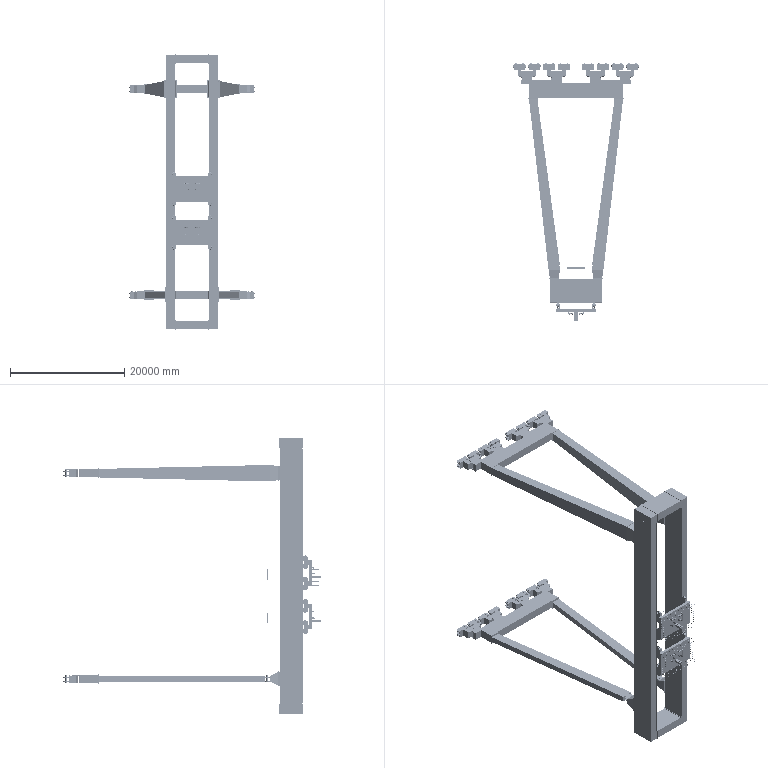Assembly | SolidWorks | mm | 212 component files | 216 solids | 10442 faces | box 22000.01 x 45009.52 x 48200 mm | volume 247326678833 mm3 | plane 6096 | cylinder 3432 | torus 512 | spline 402 | commonest cylinder face diameters 40 x1936 300 x592 200 x396 1000 x192 160 x88 80 x48 10 x32 700 x32
Bill of materials:
EndBeam | 2 |  | Rectangular box-shaped enclosure with a solid top and sides, and a thin plate at each end that sticks out a little past the body outline. One end plate has a row of small holes around its edge and a rounded-rectangle cutout in the middle.
FlexibleLegGenuine | 2 |  | Long, straight beam with a rectangular cross-section. One end has a wider rectangular plate with holes around its edge. The other end has two parallel flat tabs with rounded ends and a hole in each, like a clevis.
FlexibleLegPinAxis | 2 |  | Plain solid cylinder with flat ends.
FlexibleLegSaddleBody | 2 |  | Tapered transition body. The large end is a flat rectangular flange with holes around its edge and a rounded-rectangle opening. The body narrows to the other end, which carries three parallel lug plates with rounded tops and a through hole, like a multi-tab clevis.
16 | 2 |  | Thin, flat rectangular plate or panel with a few small slots and tabs near its centre. A wireframe-only rectangular box with evenly spaced cross lines sits on one side of it.
18 | 4 |  | Solid rectangular bar with a slightly larger, thin rectangular plate at one end.
20 | 8 |  | Clevis- or fork-shaped part: two parallel flat side plates with rounded ends, joined by a cross pin near the rounded end. The other end of the plates attaches to a flat rectangular base plate.
21 | 2 |  | Flat rectangular panel with narrow upright end strips. The strips run the full height and stick out past the panel on one face and at the top and bottom.
22 | 4 |  | Cylindrical roller or tube with a flanged collar near each end. An arm on each end runs out sideways and ends in a small rectangular block. From the end, one side is round and the other is a straight arm with a widened tip, like a keyhole.
27 | 2 |  | Wire form with two side-by-side helical coil sections joined by a U-shaped loop. A long straight leg runs from each coil and ends in a small coiled end, like a double torsion spring.
28 | 2 |  | Wire form with two side-by-side helical coil sections joined by a U-shaped loop. A long straight leg runs from each coil and ends in a small coiled end, like a double torsion spring.
Part15 | 16 |  | Grooved disc, like a pulley or spool: a short cylinder with a centre bore and a deep groove around its outside between two equal side flanges.
Part16 | 8 |  | Thin-walled U-channel bracket with two parallel side walls joined by a base web; one wall carries two round through-holes and a raised rectangular block or step on the outer face of the web.
Part17 | 16 |  | Plain solid cylinder (round rod segment) with flat ends.
LowerCrossbeam | 2 |  | Long straight rectangular box-section body with a thin flange plate at each end; each flange has a row of small holes around its edge and a U-shaped raised or recessed feature on its face.
MainBeam | 2 |  | Tall, slender rectangular bar or plate with small steps, tabs or notches along its long edges and near its ends.
RigidLeg | 2 |  | Long hollow rectangular duct section that tapers along its length, with a flat flange at each end; the flanges have perimeter holes and the larger end shows nested internal walls or vanes.
RigidLegSaddleBody | 2 |  | Short, flanged, hollow rectangular transition piece with tapered sides and bolt-hole flanges at both ends; looking through it shows a rounded-rectangle opening crossed by horizontal bars.
10 | 8 |  | Headed cylindrical pin: a plain round shank with a larger, thin, flat circular head at one end.
7 | 8 |  | Solid block with a flat top, vertical sides and a faceted underside (flat bottom with angled faces at each end), with slightly rounded edges and a single vertical round hole at the centre.
9 | 64 |  | Flat annular washer-like ring with a central round hole and rounded outer and inner edges.
Part12 | 16 |  | C-shaped bracket with two parallel flanges extending from a back body: the top flange has two round holes and the lower flange has a visible hole. A rectangular rib on the back body and a short cylindrical boss or pin sticking out at its top and bottom.
Part13 | 4 |  | Elongated thin-walled C-channel bracket with angled, tapered mounting tabs at each end, each tab with one small round hole; the channel has a small step on its underside.
Part14 | 32 |  | Plain solid cylinder (rod or pin) with flat ends, longer than its diameter.
Mates:
1. coincident | MainBeam-1 face at (3551.042, 16068.918, 30073.003) dir (0.0000002, 0, 1) | MainBeam-2 face at (-4068.958, 16068.918, 30073.004) dir (0.0000002, 0, 1)
2. distance | MainBeam-1 face at (2801.042, 18068.918, 30073.003) dir (-1, 0, 0.0000002) | MainBeam-2 face at (-3318.968, 18068.918, -17926.996) dir (1, 0, -0.0000002)
3. coincident | MainBeam-1 face at (4301.042, 18068.918, 30073.003) dir (0, 1, 0) | MainBeam-2 face at (-4818.968, 18068.918, -17926.995) dir (0, 1, 0)
4. width | EndBeam-1 face at (-3158.958, 16068.918, 29323.004) dir (-1, 0, 0.0000002) | EndBeam-1 face at (2641.042, 16068.918, 29323.003) dir (1, 0, -0.0000002) | MainBeam-2 face at (-3318.968, 18068.918, -17926.996) dir (1, 0, -0.0000002) | MainBeam-1 face at (2801.042, 18068.918, 30073.003) dir (-1, 0, 0.0000002)
5. coincident | EndBeam-1 face at (-3143.958, 18068.918, 30073.004) dir (0.0000002, 0, 1) | MainBeam-1 face at (3551.042, 16068.918, 30073.003) dir (0.0000002, 0, 1)
6. coincident | EndBeam-1 face at (-3143.958, 18068.918, 30073.004) dir (0, 1, 0) | MainBeam-1 face at (4301.042, 18068.918, 30073.003) dir (0, 1, 0)
7. coincident | RigidLegSaddleBody-1 face at (-4068.959, 18218.918, 24073.004) dir (0, -1, 0) | MainBeam-2 face at (-4068.963, 18218.918, 6073.004) dir (0, 1, 0)
8. width | RigidLegSaddleBody-1 face at (-3218.96, 18278.918, 22773.004) dir (1, 0, -0.0000002) | RigidLegSaddleBody-1 face at (-4918.959, 18278.918, 25373.005) dir (-1, 0, 0.0000002) | MainBeam-2 face at (-4918.96, 18218.918, 22758.005) dir (-1, 0, 0.0000002) | MainBeam-2 face at (-3218.959, 18218.918, 25388.004) dir (1, 0, -0.0000002)
9. width | RigidLegSaddleBody-1 face at (-3218.959, 18278.918, 25388.004) dir (0.0000002, 0, 1) | RigidLegSaddleBody-1 face at (-4918.96, 18278.918, 22758.005) dir (-0.0000002, 0, -1) | MainBeam-2 face at (-3218.96, 18218.918, 22758.004) dir (-0.0000002, 0, -1) | MainBeam-2 face at (-4918.959, 18218.918, 25388.005) dir (0.0000002, 0, 1)
10. width | RigidLeg-1 face at (-2968.959, 19718.918, 25623.004) dir (0.0000002, 0, 1) | RigidLeg-1 face at (-5168.96, 19718.918, 22523.005) dir (-0.0000002, 0, -1) | RigidLegSaddleBody-1 face at (-2968.96, 19658.918, 22523.004) dir (-0.0000002, 0, -1) | RigidLegSaddleBody-1 face at (-5168.959, 19658.918, 25623.005) dir (0.0000002, 0, 1)
11. width | RigidLeg-1 face at (-5168.959, 19718.918, 25623.005) dir (-1, 0, 0.0000002) | RigidLeg-1 face at (-2968.96, 19718.918, 22523.004) dir (1, 0, -0.0000002) | RigidLegSaddleBody-1 face at (-5168.96, 19658.918, 22523.005) dir (-1, 0, 0.0000002) | RigidLegSaddleBody-1 face at (-2968.959, 19658.918, 25623.004) dir (1, 0, -0.0000002)
12. coincident | RigidLeg-1 face at (-7752.496, 19718.918, 24073.005) dir (0, -1, 0) | RigidLegSaddleBody-1 face at (-4068.959, 19718.918, 24073.004) dir (0, 1, 0)
13. width | FlexibleLegGenuine-2 face at (-7752.504, 49658.918, -12426.995) dir (-0.0000002, 0, -1) | FlexibleLegGenuine-2 face at (-7752.503, 49658.918, -11426.995) dir (0.0000002, 0, 1) | FlexibleLegSaddleBody-1 face at (-4068.967, 18762.883, -12901.694) dir (-0.00000018, 0.4447, -0.8957) | FlexibleLegSaddleBody-1 face at (-4068.966, 18762.883, -10952.297) dir (0.00000018, 0.4447, 0.8957)
14. tangent | FlexibleLegSaddleBody-1 face at (-4068.967, 20018.918, -11506.996) dir (0.0000002, 0, 1) r 600 | FlexibleLegGenuine-2 face at (-7752.503, 20618.918, -11926.995) dir (0, -1, 0)
15. concentric | FlexibleLegSaddleBody-1 edge at (-4068.967, 20198.918, -11966.996) dir (0.0000002, 0, 1) r 200 | FlexibleLegGenuine-2 edge at (-4068.967, 20198.918, -11736.996) dir (-0.0000002, 0, -1) r 200
16. parallel | MainBeam-2 face at (-4068.968, 16068.918, -17926.996) dir (-0.0000002, 0, -1) | FlexibleLegGenuine-2 face at (-7752.504, 49658.918, -12426.995) dir (-0.0000002, 0, -1)
17. parallel | RigidLeg-1 face at (-7752.496, 49718.918, 24073.005) dir (0, 1, 0) | assembly plane at (0, 0, 0) dir (0, 1, 0)
18. coincident | FlexibleLegSaddleBody-1 face at (-4068.967, 18218.918, -11926.996) dir (0, -1, 0) | MainBeam-2 face at (-4068.963, 18218.918, 6073.004) dir (0, 1, 0)
19. width | FlexibleLegSaddleBody-1 face at (-4918.966, 18218.918, -10611.995) dir (-1, 0, 0.0000002) | FlexibleLegSaddleBody-1 face at (-3218.967, 18218.918, -13241.996) dir (1, 0, -0.0000002) | MainBeam-2 face at (-3218.967, 18218.918, -13241.996) dir (1, 0, -0.0000002) | MainBeam-2 face at (-4918.966, 18218.918, -10611.995) dir (-1, 0, 0.0000002)
20. width | FlexibleLegSaddleBody-1 face at (-4918.967, 18218.918, -13241.995) dir (-0.0000002, 0, -1) | FlexibleLegSaddleBody-1 face at (-3218.966, 18218.918, -10611.996) dir (0.0000002, 0, 1) | MainBeam-2 face at (-4918.967, 18218.918, -13241.995) dir (-0.0000002, 0, -1) | MainBeam-2 face at (-3218.966, 18218.918, -10611.996) dir (0.0000002, 0, 1)
21. coincident | FlexibleLegSaddleBody-1 edge at (-4068.967, 20198.918, -12426.996) dir (-0.0000002, 0, -1) r 200 | FlexibleLegPinAxis-1 face at (-4068.967, 20198.918, -12526.996) dir (0.0000002, 0, 1) r 200
22. width | FlexibleLegPinAxis-1 face at (-4068.967, 20198.918, -12526.996) dir (-0.0000002, 0, -1) | FlexibleLegPinAxis-1 face at (-4068.967, 20198.918, -11326.996) dir (0.0000002, 0, 1) | FlexibleLegSaddleBody-1 face at (-5068.967, 19778.918, -11426.995) dir (0.0000002, 0, 1) | FlexibleLegSaddleBody-1 face at (-3068.967, 19778.918, -12426.996) dir (-0.0000002, 0, -1)
23. coincident | RigidLeg-1 face at (-7752.496, 49718.918, 24073.005) dir (0, 1, 0) | LowerCrossbeam-2 face at (-258.959, 49718.918, 24073.004) dir (0, -1, 0)
24. coincident | LowerCrossbeam-2 face at (-8502.494, 52378.918, 24823.005) dir (0, 1, 0) | assembly face at (8891.426, 52779.524, 24005.005) dir (0, -1, 0)
25. width | RunningMechanism-1/7-1 face at (8341.041, 54548.441, 24723.002) dir (0.0000002, 0, 1) | RunningMechanism-1/7-1 face at (8341.04, 54548.441, 23423.002) dir (-0.0000002, 0, -1) | LowerCrossbeam-2 face at (-258.96, 51128.918, 23323.004) dir (-0.0000002, 0, -1) | LowerCrossbeam-2 face at (-258.959, 51128.918, 24823.004) dir (0.0000002, 0, 1)
26. coincident | LowerCrossbeam-2 face at (-8502.494, 52378.918, 24823.005) dir (0, 1, 0) | RunningMechanism-1/Part13-1 face at (5741.04, 52378.918, 23373.003) dir (0, -1, 0)
27. distance | assembly plane at (-258.964, 0, 0.000051) dir (1, 0, -0.0000002) | RunningMechanism-1/Part13-1 face at (4741.04, 52428.918, 23373.003) dir (-1, 0, 0.0000002)
28. tangent | MainBeam-1 face at (2801.042, 13918.918, 30073.003) dir (0, -1, 0) | LiftingAndOperatingMechanism-1/Part15-1 face at (2726.037, 13568.918, 4082.152) dir (-1, 0, 0.0000002) r 350
29. width | LiftingAndOperatingMechanism-1/Part16-1 face at (3126.037, 13443.918, 4782.152) dir (1, 0, -0.0000002) | LiftingAndOperatingMechanism-1/Part16-1 face at (2626.037, 13443.918, 4782.152) dir (-1, 0, 0.0000002) | MainBeam-1 face at (2801.042, 18068.918, 30073.003) dir (-1, 0, 0.0000002) | MainBeam-1 face at (2951.042, 14068.918, 30073.003) dir (1, 0, -0.0000002)
30. parallel | MainBeam-1 face at (4301.042, 14068.918, 30073.003) dir (0, -1, 0) | LiftingAndOperatingMechanism-1/16-1 face at (-258.963, 12918.918, 6632.153) dir (0, 1, 0)
31. width | LiftingAndOperatingMechanism-2/Part16-1 face at (3126.035, 13443.918, -2871.046) dir (1, 0, -0.0000002) | LiftingAndOperatingMechanism-2/Part16-1 face at (2626.035, 13443.918, -2871.046) dir (-1, 0, 0.0000002) | MainBeam-1 face at (2801.042, 18068.918, 30073.003) dir (-1, 0, 0.0000002) | MainBeam-1 face at (2951.042, 14068.918, 30073.003) dir (1, 0, -0.0000002)
32. tangent | MainBeam-2 face at (-3318.968, 13918.918, -17926.996) dir (0, -1, 0) | LiftingAndOperatingMechanism-2/Part15-4 face at (-3243.965, 13568.918, -3571.045) dir (1, 0, -0.0000002) r 350
33. coincident | FlexibleLegGenuine-2 face at (-6902.504, 49718.918, -12776.995) dir (-0.0000002, 0, -1) | LowerCrossbeam-3 face at (-8602.502, 49718.918, -12776.995) dir (-0.0000002, 0, -1)
34. coincident | 16-1 edge at (1000, 480, -300) dir (-1, 0, 0) | 18-2 edge at (1000, 480, -300) dir (-1, 0, 0)
35. coincident | 16-1 edge at (600, 480, -300) dir (0, 0, 1) | 18-2 edge at (600, 480, -300) dir (0, 0, 1)
36. coincident | 16-1 edge at (0, 480, 670) dir (1, 0, 0) | 20-2 edge at (0, 480, 670) dir (1, 0, 0)
37. coincident | 16-1 edge at (200, 480, 670) dir (0, 0, -1) | 20-2 edge at (200, 480, 670) dir (0, 0, -1)
38. coincident | 16-1 edge at (-1000, 480, 1340) dir (1, 0, 0) | 22-1 edge at (-1000, 480, 1340) dir (1, 0, 0)
39. coincident | 16-1 edge at (-1000, 480, 1260) dir (0, 0, 1) | 22-1 edge at (-1000, 480, 1260) dir (0, 0, 1)
40. coincident | 16-1 edge at (430, 480, 1280) dir (1, 0, 0) | 20-1 edge at (280, 480, 1280) dir (1, 0, 0)
41. coincident | 16-1 edge at (480, 480, 1280) dir (0, 0, -1) | 20-1 edge at (480, 480, 1280) dir (0, 0, -1)
42. concentric | 22-1 face at (-900, 820, 520) dir (0, 0, 1) r 130 | 27-1 sketch segment at (-900, 820, 525) dir (0, 0, 1) r 135
43. concentric | 20-1 face at (380, 910, 1255) dir (0, 0, -1) r 40 | 27-1 sketch segment at (380, 910, 525) dir (0, 0, 1) r 45
44. tangent | 22-1 face at (-900, 820, 520) dir (0, 0, 1) | 27-1 face at (-900, 955, 525) dir (1, 0, 0) r 5
45. concentric | 22-2 face at (-900, 820, -1280) dir (0, 0, 1) r 130 | 28-1 sketch segment at (-900, 820, -1225) dir (0, 0, 1) r 135
46. concentric | 20-4 face at (380, 910, -1105) dir (0, 0, -1) r 40 | 28-1 sketch segment at (380, 910, -1225) dir (0, 0, 1) r 45
47. tangent | 22-2 face at (-900, 820, -520) dir (0, 0, -1) | 28-1 face at (-900, 955, -525) dir (1, 0, 0) r 5
48. concentric | 21-1 sketch segment at (144.999, -7090.265, 603.75) dir (0, 1, 0) r 5 | LiftingAndOperatingMechanism sketch segment at (144.999, -7090.265, 603.75) dir (0, -1, 0) r 5
49. concentric | 21-1 sketch segment at (425, -7090.265, 1146.25) dir (0, 1, 0) r 5 | LiftingAndOperatingMechanism sketch segment at (425, -7090.265, 1146.25) dir (0, -1, 0) r 5
50. coincident | 21-1 face at (524.311, -7090.265, -0.000113) dir (0, 1, 0) | LiftingAndOperatingMechanism sketch segment at (425, -7090.265, 1146.25) dir (0, -1, 0) r 5
51. coincident | 16-1 face at (0, 0, 0) dir (0, -1, 0) | Part16-1 face at (1450, 0, -2885) dir (0, 1, 0)
52. coincident | 16-1 face at (2250, 500, -3585) dir (1, 0, 0) | Part16-1 face at (2250, -100, -2885) dir (1, 0, 0)
53. width | Part15-1 face at (2550, -150, -2985) dir (0, 0, 1) | Part15-1 face at (2550, -650, -3285) dir (0, 0, -1) | Part16-1 face at (1850, -525, -3385) dir (0, 0, -1) | Part16-1 face at (1850, -525, -2885) dir (0, 0, 1)
54. concentric | Part15-1 face at (2550, -650, -2985) dir (0, 0, 1) r 500 | Part16-1 face at (2550, -650, -3385) dir (0, 0, 1) r 150
55. distance | Part16-1 face at (1850, -525, -3385) dir (0, 0, -1) | 16-1 face at (-2250, 500, -3585) dir (0, 0, -1)
56. concentric | Part16-1 face at (1150, -650, -3385) dir (0, 0, 1) r 153.74 | Part15-3 face at (1150, -650, -3285) dir (0, 0, -1) r 500
57. width | Part15-3 face at (1150, -1150, -3285) dir (0, 0, -1) | Part15-3 face at (1150, -650, -2985) dir (0, 0, 1) | Part16-1 face at (1850, -525, -2885) dir (0, 0, 1) | Part16-1 face at (1850, -525, -3385) dir (0, 0, -1)
58. concentric | Part16-1 face at (2550, -650, -3385) dir (0, 0, 1) r 150 | Part17-1 face at (2550, -650, -2835) dir (0, 0, -1) r 150
59. width | Part17-1 face at (2550, -650, -2835) dir (0, 0, 1) | Part17-1 face at (2550, -650, -3435) dir (0, 0, -1) | Part16-1 face at (1850, -525, -3385) dir (0, 0, -1) | Part16-1 face at (1850, -525, -2885) dir (0, 0, 1)
60. concentric | Part16-1 face at (1150, -650, -3385) dir (0, 0, 1) r 153.74 | Part17-2 face at (1150, -650, -2835) dir (0, 0, -1) r 150
61. width | Part17-2 face at (1150, -650, -3435) dir (0, 0, -1) | Part17-2 face at (1150, -650, -2835) dir (0, 0, 1) | Part16-1 face at (1850, -525, -2885) dir (0, 0, 1) | Part16-1 face at (1850, -525, -3385) dir (0, 0, -1)
62. concentric | 7-1 face at (0, -600, -650) dir (0, 0, 1) r 150 | 10-1 face at (0, -600, 750) dir (0, 0, -1) r 150
63. parallel | 7-1 face at (0, -1250, 650) dir (0, 0, 1) | Part12-1 face at (-1300, -1975, -650) dir (0, 0, -1)
64. coincident | 7-1 edge at (-1600, -499.104, -650) dir (0, -1, 0) | Part12-1 face at (-1600, -1550, 650) dir (-1, 0, 0)
65. concentric | 9-1 face at (-1900, -2100, 450) dir (0, 0, -1) r 150 | Part12-1 face at (-1900, -2100, -650) dir (0, 0, 1) r 150
66. coincident | 7-1 face at (0, -1250, 650) dir (0, 0, 1) | Part12-1 face at (-1300, -1975, 650) dir (0, 0, 1)
67. concentric | 9-5 face at (-700, -2100, 450) dir (0, 0, -1) r 150 | Part12-1 face at (-700, -2100, -650) dir (0, 0, 1) r 150
68. coincident | 9-1 face at (-1900, -2100, 450) dir (0, 0, 1) | 9-5 face at (-700, -2100, 450) dir (0, 0, 1)
69. coincident | 7-1 face at (-1600, -1250, 650) dir (0, -1, 0) | Part12-1 face at (-1600, -1250, 650) dir (0, 1, 0)
70. width | Part13-1 face at (2600, 1206.955, -700) dir (0, 0, -1) | Part13-1 face at (2600, 1206.955, 700) dir (0, 0, 1) | 7-1 face at (0, -1250, 650) dir (0, 0, 1) | 7-1 face at (0, -1250, -650) dir (0, 0, -1)
71. width | Part13-1 face at (6157.744, 869.523, -700) dir (1, 0, 0) | Part13-1 face at (-957.744, 1206.955, -700) dir (-1, 0, 0) | 7-1 face at (-1600, -413.97, 650) dir (-1, 0, 0) | 7-2 face at (6800, -413.97, -650) dir (1, 0, 0)
72. concentric | Part12-4 face at (4500, -2100, -650) dir (0, 0, 1) r 150 | 9-17 face at (4500, -2100, 450) dir (0, 0, -1) r 150
73. width | Part12-3 face at (6500, -1975, -650) dir (0, 0, -1) | Part12-3 face at (6500, -1975, 650) dir (0, 0, 1) | 9-13 face at (7100, -2100, 450) dir (0, 0, 1) | 9-19 face at (7100, -2100, -450) dir (0, 0, -1)
74. concentric | 9-1 face at (-1900, -2100, 450) dir (0, 0, -1) r 150 | Part14-1 face at (-1900, -2100, -700) dir (0, 0, 1) r 150
75. width | Part14-1 face at (-1900, -2100, -700) dir (0, 0, -1) | Part14-1 face at (-1900, -2100, 700) dir (0, 0, 1) | Part12-1 face at (-1300, -1975, 650) dir (0, 0, 1) | Part12-1 face at (-1300, -1975, -650) dir (0, 0, -1)
76. concentric | 9-5 face at (-700, -2100, 450) dir (0, 0, -1) r 150 | Part14-2 face at (-700, -2100, -700) dir (0, 0, 1) r 150
77. width | Part14-2 face at (-700, -2100, 700) dir (0, 0, 1) | Part14-2 face at (-700, -2100, -700) dir (0, 0, -1) | Part12-1 face at (-1300, -1975, -650) dir (0, 0, -1) | Part12-1 face at (-1300, -1975, 650) dir (0, 0, 1)